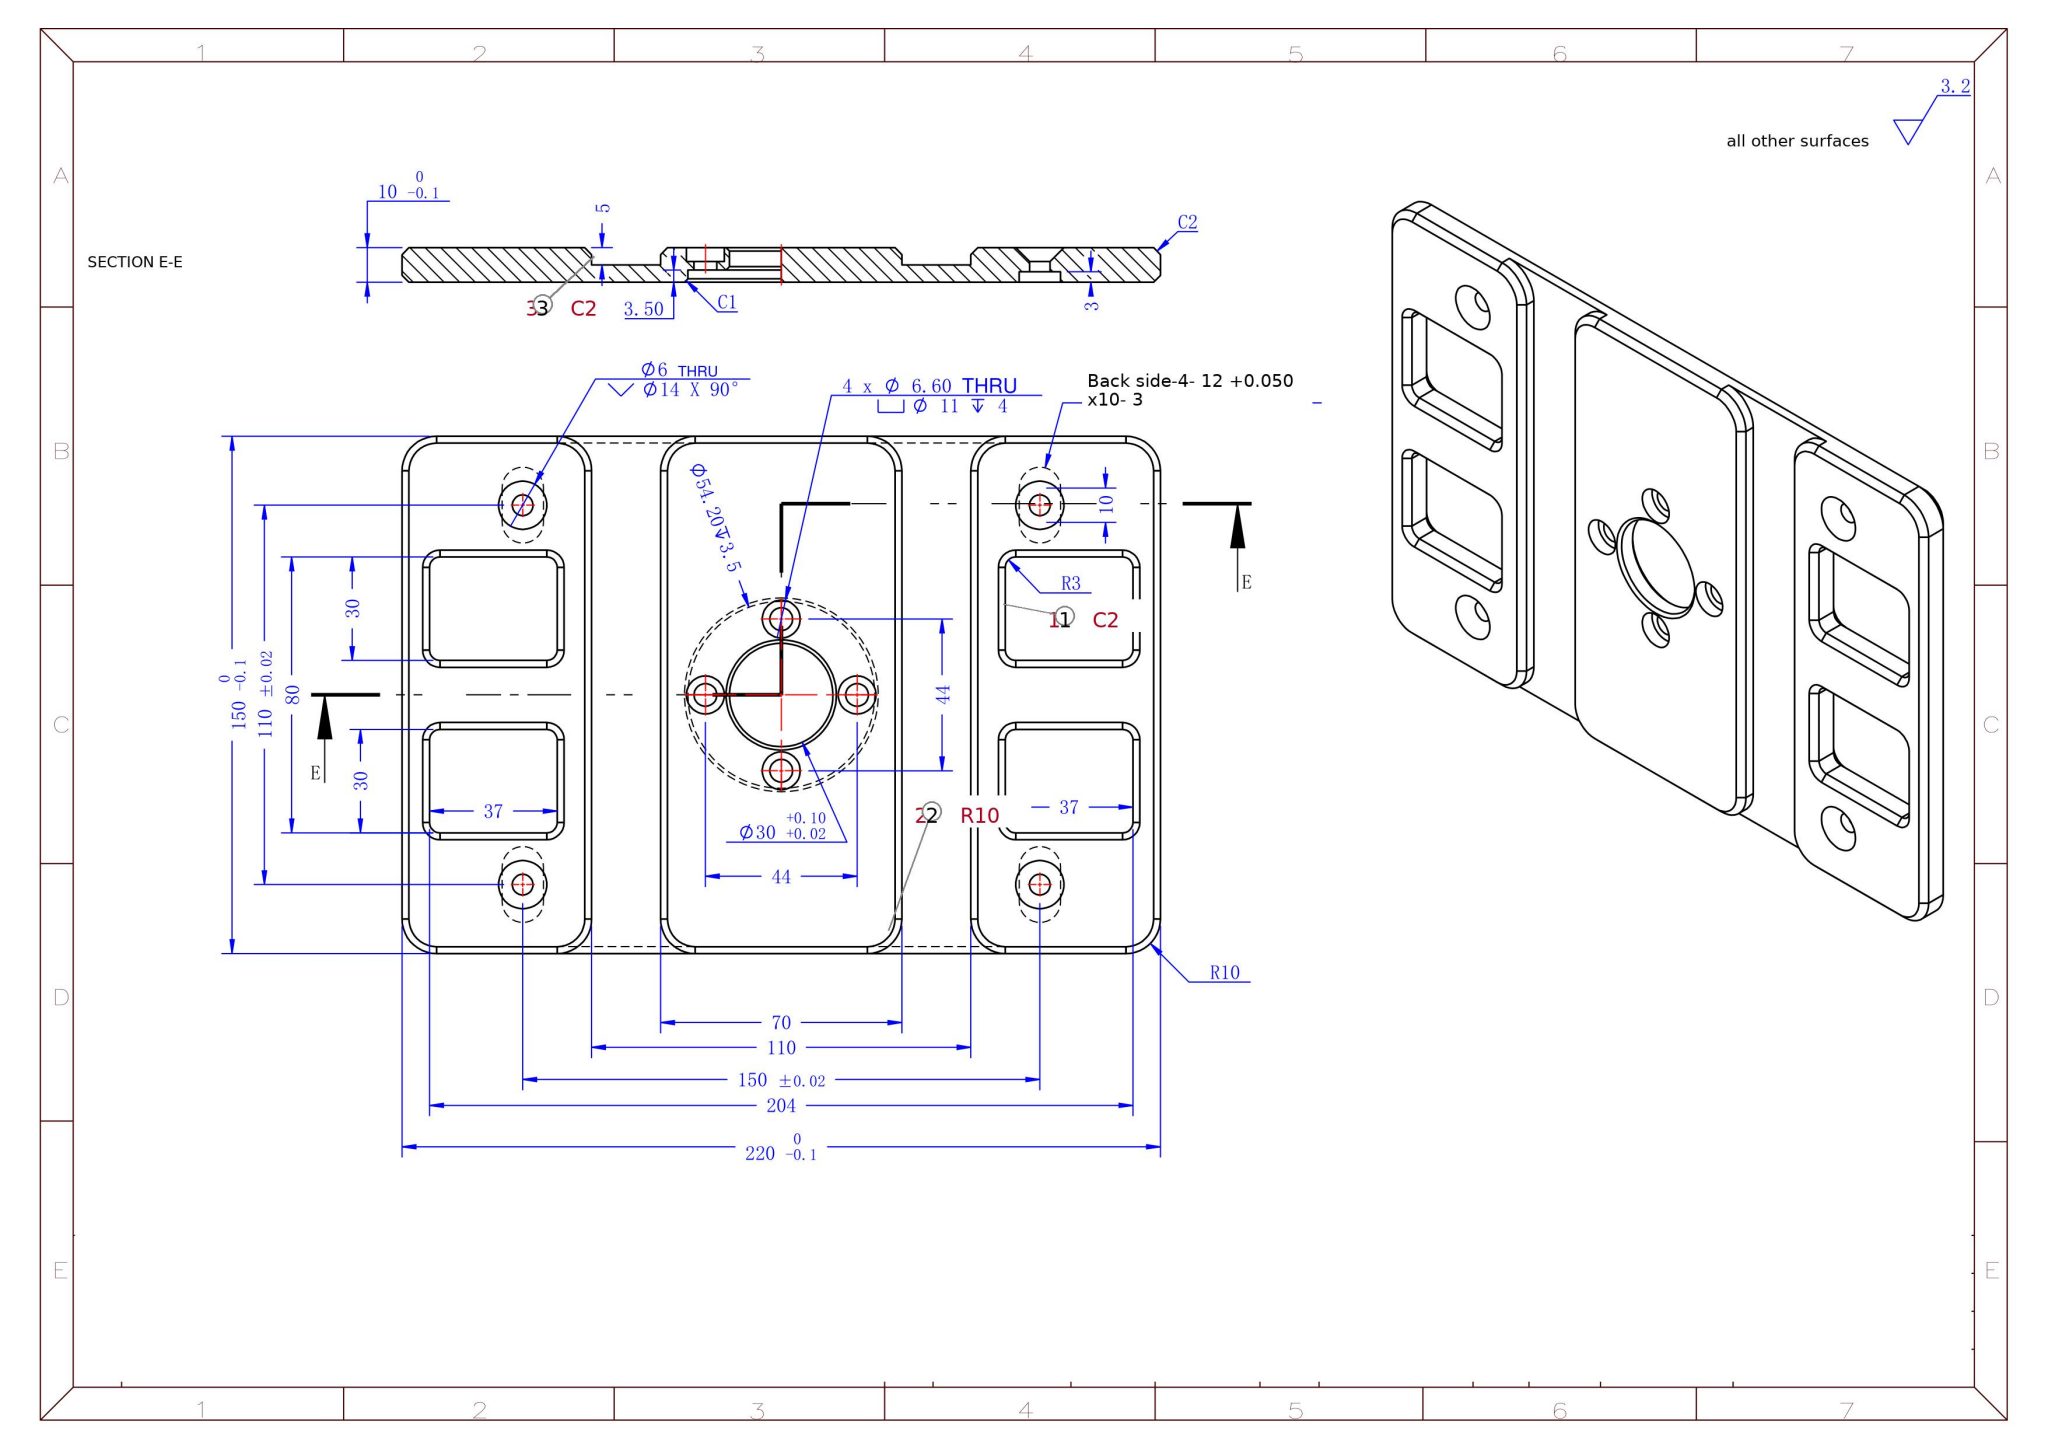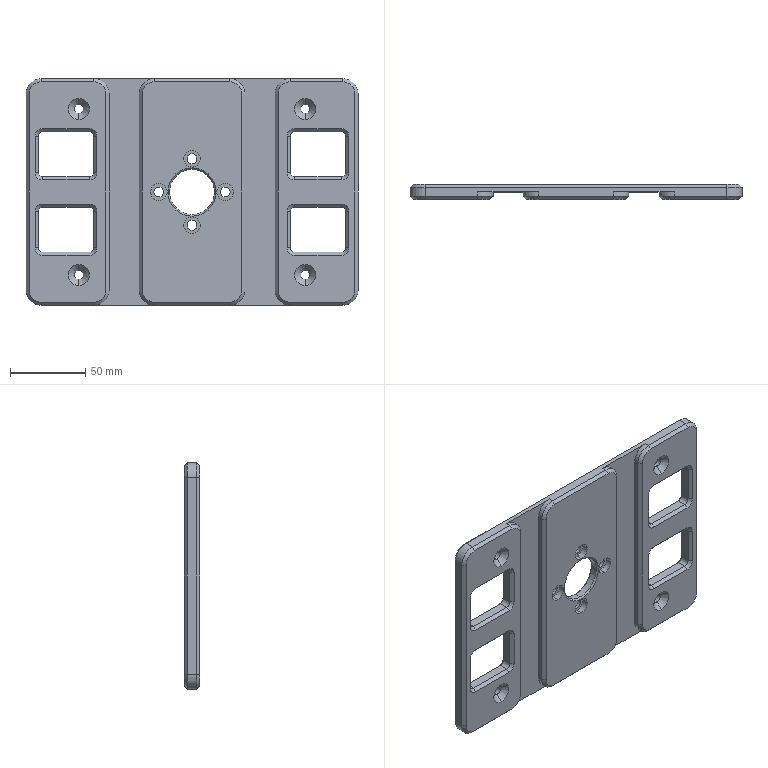Part | SolidWorks | mm | 1 solid | 225 faces | box 220 x 10 x 150 mm | volume 229059 mm3 | plane 95 | cylinder 68 | cone 62 | commonest cylinder face diameters 6 x24 12 x12 20 x12 11 x8 6.6 x8 30 x2 54.2 x2
build123d program:
from build123d import *

# Parameters (mm, degrees)
SKETCH1_W                                       = 220
SKETCH1_H                                       = 150
BOSS_EXTRUDE1_DEPTH                             = 10
SKETCH2_R                                       = 6
CUT_EXTRUDE1_DEPTH                              = 3
SKETCH3_R                                       = 3
CUT_EXTRUDE2_DEPTH                              = 134.51
SKETCH6_R                                       = 27.1
CUT_EXTRUDE4_DEPTH                              = 3.5
SKETCH7_R                                       = 15
CUT_EXTRUDE5_DEPTH                              = 134.294
M6_HEX_SOCKET_HEAD_CAP_SCREW_CBORE1_D           = 6.6
M6_HEX_SOCKET_HEAD_CAP_SCREW_CBORE1_CBORE_D     = 11
M6_HEX_SOCKET_HEAD_CAP_SCREW_CBORE1_CBORE_DEPTH = 4
SKETCH11_W                                      = 20
SKETCH11_H                                      = 150
CUT_EXTRUDE6_DEPTH                              = 5
CUT_EXTRUDE8_DEPTH                              = 134.319
SKETCH14_W                                      = 37
SKETCH14_H                                      = 30
CUT_EXTRUDE9_DEPTH                              = 134.51
FILLET1_R                                       = 10
FILLET2_R                                       = 3
CHAMFER1_SIZE                                   = 2
CHAMFER2_SIZE                                   = 4
CHAMFER3_SIZE                                   = 1


with BuildPart() as part:
    # Sketch1 → Boss-Extrude1 (new body)
    with BuildSketch(Plane(origin=(0, 0, 0), x_dir=(1, 0, 0), z_dir=(0, 1, 0))):
        Rectangle(SKETCH1_W, SKETCH1_H)
    extrude(amount=BOSS_EXTRUDE1_DEPTH)

    # Sketch2 → Cut-Extrude1 (cut)
    with BuildSketch(Plane(origin=(0, 10, 0), x_dir=(1, 0, 0), z_dir=(0, 1, 0))):
        with Locations(Location((-75, 55, 0), (0, 0, 270))):
            Circle(SKETCH2_R)
        with Locations(Location((75, 55, 0), (0, 0, 270))):
            Circle(SKETCH2_R)
        with Locations(Location((75, -55, 0), (0, 0, 270))):
            Circle(SKETCH2_R)
        with Locations(Location((-75, -55, 0), (0, 0, 270))):
            Circle(SKETCH2_R)
    extrude(amount=-CUT_EXTRUDE1_DEPTH, mode=Mode.SUBTRACT)

    # Sketch3 → Cut-Extrude2 (cut, through all)
    with BuildSketch(Plane.XZ):
        with Locations(Location((-75, 55, 0), (0, 0, 270))):
            Circle(SKETCH3_R)
        with Locations(Location((-75, -55, 0), (0, 0, 270))):
            Circle(SKETCH3_R)
        with Locations(Location((75, -55, 0), (0, 0, 270))):
            Circle(SKETCH3_R)
        with Locations(Location((75, 55, 0), (0, 0, 270))):
            Circle(SKETCH3_R)
    extrude(amount=-CUT_EXTRUDE2_DEPTH, mode=Mode.SUBTRACT)

    # Sketch6 → Cut-Extrude4 (cut)
    with BuildSketch(Plane(origin=(0, 10, 0), x_dir=(1, 0, 0), z_dir=(0, 1, 0))):
        with Locations(Location((0, 0, 0), (0, 0, 270))):
            Circle(SKETCH6_R)
    extrude(amount=-CUT_EXTRUDE4_DEPTH, mode=Mode.SUBTRACT)

    # Sketch7 → Cut-Extrude5 (cut, through all)
    with BuildSketch(Plane(origin=(0, 6.5, 0), x_dir=(1, 0, 0), z_dir=(0, 1, 0))):
        with Locations(Location((0, 0, 0), (0, 0, 270))):
            Circle(SKETCH7_R)
    extrude(amount=-CUT_EXTRUDE5_DEPTH, mode=Mode.SUBTRACT)

    # M6 Hex Socket Head Cap Screw CBORE1 (through all)
    with Locations(Plane(origin=(0, 0, 0), x_dir=(-1, 0, 0), z_dir=(0, -1, 0))):
        with Locations((0, -22), (0, 22), (22, 0), (-22, 0)):
            CounterBoreHole(M6_HEX_SOCKET_HEAD_CAP_SCREW_CBORE1_D / 2, M6_HEX_SOCKET_HEAD_CAP_SCREW_CBORE1_CBORE_D / 2, M6_HEX_SOCKET_HEAD_CAP_SCREW_CBORE1_CBORE_DEPTH)

    # Sketch11 → Cut-Extrude6 (cut)
    with BuildSketch(Plane.XZ):
        with Locations((-45, 0)):
            Rectangle(SKETCH11_W, SKETCH11_H)
        with Locations((45, 0)):
            Rectangle(SKETCH11_W, SKETCH11_H)
    extrude(amount=-CUT_EXTRUDE6_DEPTH, mode=Mode.SUBTRACT)

    # Sketch13 → Cut-Extrude8 (cut, through all)
    with BuildSketch(Plane(origin=(0, 7, 0), x_dir=(1, 0, 0), z_dir=(0, 1, 0))):
        with BuildLine():
            Line((-69, 60), (-69, 50))
            ThreePointArc((-69, 50), (-75, 44), (-81, 50))
            Line((-81, 50), (-81, 60))
            ThreePointArc((-81, 60), (-75, 66), (-69, 60))
        make_face()
        with BuildLine():
            Line((81, 60), (81, 50))
            ThreePointArc((81, 50), (75, 44), (69, 50))
            Line((69, 50), (69, 60))
            ThreePointArc((69, 60), (75, 66), (81, 60))
        make_face()
        with BuildLine():
            Line((81, -50), (81, -60))
            ThreePointArc((81, -60), (75, -66), (69, -60))
            Line((69, -60), (69, -50))
            ThreePointArc((69, -50), (75, -44), (81, -50))
        make_face()
        with BuildLine():
            Line((-69, -50), (-69, -60))
            ThreePointArc((-69, -60), (-75, -66), (-81, -60))
            Line((-81, -60), (-81, -50))
            ThreePointArc((-81, -50), (-75, -44), (-69, -50))
        make_face()
    extrude(amount=CUT_EXTRUDE8_DEPTH, mode=Mode.SUBTRACT)

    # Sketch14 → Cut-Extrude9 (cut, through all)
    with BuildSketch(Plane.XZ):
        with Locations((-83.5, 25)):
            Rectangle(SKETCH14_W, SKETCH14_H)
        with Locations((-83.5, -25)):
            Rectangle(SKETCH14_W, SKETCH14_H)
        with Locations((83.5, 25)):
            Rectangle(SKETCH14_W, SKETCH14_H)
        with Locations((83.5, -25)):
            Rectangle(SKETCH14_W, SKETCH14_H)
    extrude(amount=-CUT_EXTRUDE9_DEPTH, mode=Mode.SUBTRACT)

    # Fillet1
    fillet1_edges = [part.edges().sort_by_distance(p)[0] for p in [
        (55, 2.5, 75),
        (55, 2.5, -75),
        (35, 2.5, -75),
        (35, 2.5, 75),
        (110, 5, 75),
        (-110, 5, 75),
        (-110, 5, -75),
        (110, 5, -75),
        (-35, 2.5, 75),
        (-35, 2.5, -75),
        (-55, 2.5, -75),
        (-55, 2.5, 75),
    ]]
    fillet(fillet1_edges, radius=FILLET1_R)

    # Fillet2
    fillet2_edges = [part.edges().sort_by_distance(p)[0] for p in [
        (-102, 5, 10),
        (-102, 5, 40),
        (-65, 5, 40),
        (-65, 5, 10),
        (-102, 5, -40),
        (-102, 5, -10),
        (-65, 5, -10),
        (-65, 5, -40),
        (102, 5, 40),
        (102, 5, 10),
        (65, 5, 10),
        (65, 5, 40),
        (102, 5, -10),
        (102, 5, -40),
        (65, 5, -40),
        (65, 5, -10),
    ]]
    fillet(fillet2_edges, radius=FILLET2_R)

    # Chamfer1
    chamfer1_edges = [part.edges().sort_by_distance(p)[0] for p in [
        (-35, 0, 0),
        (0, 0, -75),
        (35, 0, 0),
        (0, 0, 75),
        (-32.071, 0, 72.071),
        (32.071, 0, 72.071),
        (32.071, 0, -72.071),
        (-32.071, 0, -72.071),
        (82.5, 0, -75),
        (-82.5, 0, -75),
        (0, 10, -75),
        (-55, 0, 0),
        (-82.5, 0, 75),
        (-110, 0, 0),
        (-107.071, 0, -72.071),
        (-107.071, 0, 72.071),
        (-57.929, 0, 72.071),
        (-57.929, 0, -72.071),
        (55, 0, 0),
        (82.5, 0, 75),
        (110, 0, 0),
        (107.071, 0, -72.071),
        (107.071, 0, 72.071),
        (57.929, 0, 72.071),
        (57.929, 0, -72.071),
        (0, 10, 75),
        (110, 10, 0),
        (-110, 10, 0),
        (107.071, 10, -72.071),
        (-107.071, 10, -72.071),
        (-107.071, 10, 72.071),
        (107.071, 10, 72.071),
        (83.5, 0, 10),
        (83.5, 10, 10),
        (65, 0, 25),
        (65, 10, 25),
        (102, 0, 25),
        (102, 10, 25),
        (83.5, 0, 40),
        (83.5, 10, 40),
        (102, 0, -25),
        (102, 10, -25),
        (83.5, 0, -40),
        (83.5, 10, -40),
        (83.5, 0, -10),
        (83.5, 10, -10),
        (65, 0, -25),
        (65, 10, -25),
        (-65, 0, 25),
        (-65, 10, 25),
        (-83.5, 0, 10),
        (-83.5, 10, 10),
        (-83.5, 0, 40),
        (-83.5, 10, 40),
        (-102, 0, 25),
        (-102, 10, 25),
        (-65, 0, -25),
        (-65, 10, -25),
        (-83.5, 0, -40),
        (-83.5, 10, -40),
        (-83.5, 0, -10),
        (-83.5, 10, -10),
        (-102, 0, -25),
        (-102, 10, -25),
        (65.879, 0, 10.879),
        (65.879, 10, 10.879),
        (101.121, 0, 10.879),
        (101.121, 10, 10.879),
        (101.121, 0, 39.121),
        (101.121, 10, 39.121),
        (101.121, 0, -39.121),
        (101.121, 10, -39.121),
        (101.121, 0, -10.879),
        (101.121, 10, -10.879),
        (65.879, 0, -39.121),
        (65.879, 10, -39.121),
        (65.879, 0, -10.879),
        (65.879, 10, -10.879),
        (65.879, 0, 39.121),
        (65.879, 10, 39.121),
        (-65.879, 0, 10.879),
        (-65.879, 10, 10.879),
        (-65.879, 0, 39.121),
        (-65.879, 10, 39.121),
        (-101.121, 0, 10.879),
        (-101.121, 10, 10.879),
        (-65.879, 0, -39.121),
        (-65.879, 10, -39.121),
        (-65.879, 0, -10.879),
        (-65.879, 10, -10.879),
        (-101.121, 0, -10.879),
        (-101.121, 10, -10.879),
        (-101.121, 0, -39.121),
        (-101.121, 10, -39.121),
        (-101.121, 0, 39.121),
        (-101.121, 10, 39.121),
    ]]
    chamfer(chamfer1_edges, length=CHAMFER1_SIZE)

    # Chamfer2
    chamfer2_edges = [part.edges().sort_by_distance(p)[0] for p in [
        (-75, 0, 58),
        (-75, 0, -52),
        (75, 0, -52),
        (75, 0, 58),
    ]]
    chamfer(chamfer2_edges, length=CHAMFER2_SIZE)

    # Chamfer3
    chamfer3_edges = [part.edges().sort_by_distance(p)[0] for p in [
        (0, 10, -27.1),
        (0, 0, -15),
        (0, 6.5, -15),
    ]]
    chamfer(chamfer3_edges, length=CHAMFER3_SIZE)


solid = part.part